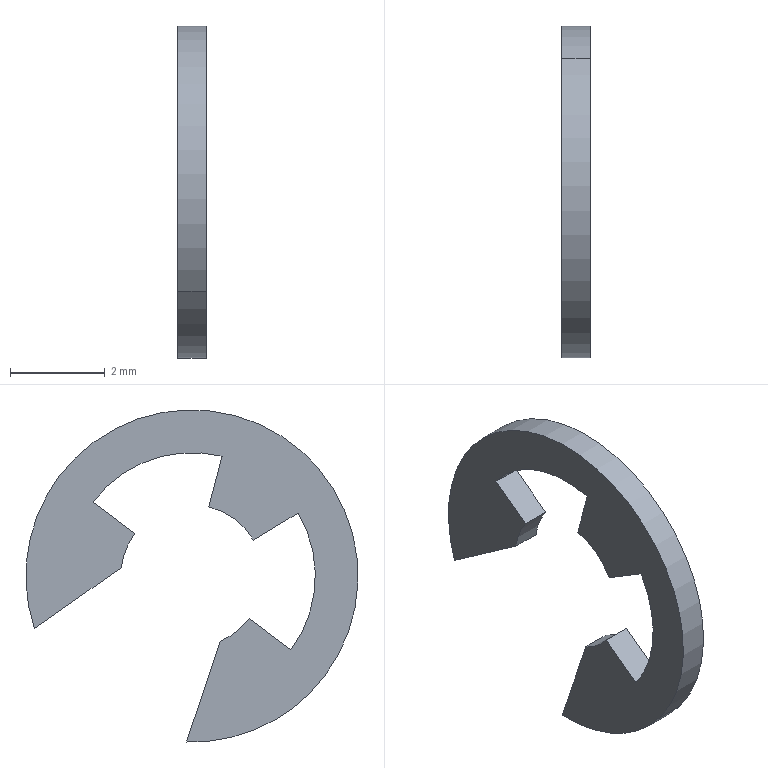Component | SolidWorks | NETWS3-1 | 1 solid | 16 faces | box 0.6 x 7 x 7 mm | volume 11 mm3 | cylinder 8 | plane 8 | commonest cylinder face diameters 7 x3 3 x3 5.2 x2
build123d program:
from build123d import *

# Parameters (mm, degrees)
BOSS_EXTRUDE1_DEPTH      = 0.3
BOSS_EXTRUDE1_DEPTH_BACK = 0.3


with BuildPart() as part:
    # Sketch1 → Boss-Extrude1 (new, two sides: drawn at the far end of the back side and taken through both)
    with BuildSketch(Plane.XY.offset(-BOSS_EXTRUDE1_DEPTH_BACK)):
        with BuildLine():
            Line((-2, -2.872), (-1.3, -0.7483))
            ThreePointArc((-1.3, -0.7483), (-1.449, -0.3873), (-1.5, 0))
            Line((-1.5, 0), (-2.6, 0))
            ThreePointArc((-2.6, 0), (-2.163, 1.442), (-1, 2.4))
            Line((-1, 2.4), (-0.587, 1.38))
            ThreePointArc((-0.587, 1.38), (0, 1.5), (0.587, 1.38))
            Line((0.587, 1.38), (1, 2.4))
            ThreePointArc((1, 2.4), (2.163, 1.442), (2.6, 0))
            Line((2.6, 0), (1.5, 0))
            ThreePointArc((1.5, 0), (1.449, -0.3873), (1.3, -0.7483))
            Line((1.3, -0.7483), (2, -2.872))
            ThreePointArc((2, -2.872), (0, 3.5), (-2, -2.872))
        make_face()
    extrude(amount=BOSS_EXTRUDE1_DEPTH + BOSS_EXTRUDE1_DEPTH_BACK)


solid = part.part

# Placed as in the assembly
solid = solid.moved(Location((-135.602, 37.141, -105.536), (126.711, 90, 0)))